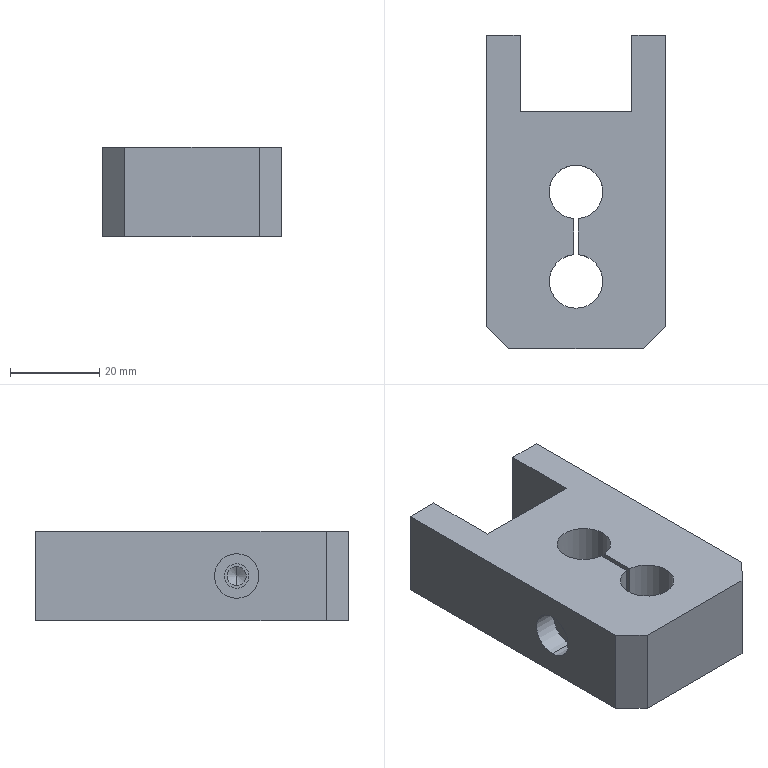Component | SolidWorks | 55-1 | 1 solid | 28 faces | box 40 x 70 x 20 mm | volume 41189 mm3 | plane 15 | cylinder 11 | cone 2 | commonest cylinder face diameters 4.2 x4 12 x3 10 x2 5.5 x2
build123d program:
from build123d import *

# Parameters (mm, degrees)
SKETCH1_W                                            = 20
SKETCH1_H                                            = 80
BOSS_EXTRUDE1_DEPTH                                  = 40
SKETCH2_R                                            = 6
CUT_EXTRUDE1_DEPTH                                   = 40
SKETCH3_W                                            = 1
SKETCH3_H                                            = 21.122
CUT_EXTRUDE2_DEPTH                                   = 40
M5_HEX_SOCKET_HEAD_CAP_SCREW_COUNTERBORE_D           = 5.5
M5_HEX_SOCKET_HEAD_CAP_SCREW_COUNTERBORE_DEPTH       = 19.5
M5_HEX_SOCKET_HEAD_CAP_SCREW_COUNTERBORE_CBORE_D     = 10
M5_HEX_SOCKET_HEAD_CAP_SCREW_COUNTERBORE_CBORE_DEPTH = 5.4
M5_TAPPED_HOLE1_D                                    = 4.2
M5_TAPPED_HOLE1_DEPTH                                = 14
M5_TAPPED_HOLE1_TIP                                  = 1.262
CHAMFER1_SIZE                                        = 5
SKETCH8_W                                            = 25
SKETCH8_H                                            = 27
CUT_EXTRUDE3_DEPTH                                   = 40
M5_TAPPED_HOLE2_D                                    = 4.2
M5_TAPPED_HOLE2_DEPTH                                = 14
M5_TAPPED_HOLE2_TIP                                  = 1.262
SKETCH11_W                                           = 40
SKETCH11_H                                           = 10
CUT_EXTRUDE4_DEPTH                                   = 61


with BuildPart() as part:
    # Sketch1 → Boss-Extrude1 (new body)
    with BuildSketch(Plane.XY):
        Rectangle(SKETCH1_W, SKETCH1_H)
    extrude(amount=BOSS_EXTRUDE1_DEPTH)

    # Sketch2 → Cut-Extrude1 (cut)
    with BuildSketch(Plane.ZY.offset(10)):
        with Locations(Location((20, -5, 0), (0, 0, 270))):
            Circle(SKETCH2_R)
        with Locations(Location((20, -25, 0), (0, 0, 270))):
            Circle(SKETCH2_R)
    extrude(amount=-CUT_EXTRUDE1_DEPTH, mode=Mode.SUBTRACT)

    # Sketch3 → Cut-Extrude2 (cut)
    with BuildSketch(Plane.ZY.offset(10)):
        with Locations((20, -14.461)):
            Rectangle(SKETCH3_W, SKETCH3_H)
    extrude(amount=-CUT_EXTRUDE2_DEPTH, mode=Mode.SUBTRACT)

    # M5 Hex Socket Head Cap Screw Counterbore
    with Locations(Plane.XY.offset(40)):
        with Locations((0, -15)):
            CounterBoreHole(M5_HEX_SOCKET_HEAD_CAP_SCREW_COUNTERBORE_D / 2, M5_HEX_SOCKET_HEAD_CAP_SCREW_COUNTERBORE_CBORE_D / 2, M5_HEX_SOCKET_HEAD_CAP_SCREW_COUNTERBORE_CBORE_DEPTH, depth=M5_HEX_SOCKET_HEAD_CAP_SCREW_COUNTERBORE_DEPTH)

    # M5 Tapped Hole1
    with Locations(Plane.XY.offset(19.5)):
        with Locations((0, -15)):
            Hole(M5_TAPPED_HOLE1_D / 2, depth=M5_TAPPED_HOLE1_DEPTH)
            with Locations((0, 0, -(M5_TAPPED_HOLE1_DEPTH + M5_TAPPED_HOLE1_TIP / 2))):  # 118° drill point
                Cone(0, M5_TAPPED_HOLE1_D / 2, M5_TAPPED_HOLE1_TIP, mode=Mode.SUBTRACT)

    # Chamfer1
    chamfer1_edges = [part.edges().sort_by_distance(p)[0] for p in [
        (0, -40, 0),
        (0, -40, 40),
    ]]
    chamfer(chamfer1_edges, length=CHAMFER1_SIZE)

    # Sketch8 → Cut-Extrude3 (cut)
    with BuildSketch(Plane.ZY.offset(10)):
        with Locations((20, 26.5)):
            Rectangle(SKETCH8_W, SKETCH8_H)
    extrude(amount=-CUT_EXTRUDE3_DEPTH, mode=Mode.SUBTRACT)

    # M5 Tapped Hole2
    with Locations(Plane(origin=(0, 13, 0), x_dir=(1, 0, 0), z_dir=(0, 1, 0))):
        with Locations((0, -20)):
            Hole(M5_TAPPED_HOLE2_D / 2, depth=M5_TAPPED_HOLE2_DEPTH)
            with Locations((0, 0, -(M5_TAPPED_HOLE2_DEPTH + M5_TAPPED_HOLE2_TIP / 2))):  # 118° drill point
                Cone(0, M5_TAPPED_HOLE2_D / 2, M5_TAPPED_HOLE2_TIP, mode=Mode.SUBTRACT)

    # Sketch11 → Cut-Extrude4 (cut, through all)
    with BuildSketch(Plane.ZY.offset(10)):
        with Locations((20, 35)):
            Rectangle(SKETCH11_W, SKETCH11_H)
    extrude(amount=-CUT_EXTRUDE4_DEPTH, mode=Mode.SUBTRACT)


solid = part.part

# Placed as in the assembly
solid = solid.moved(Location((20, -13, 100), (0, -90, 0)))
STEP:
#1=COLOUR_RGB('',0.7922,0.8196,0.9333);
#2=FILL_AREA_STYLE_COLOUR('',#1);
#3=FILL_AREA_STYLE('',(#2));
#4=SURFACE_STYLE_FILL_AREA(#3);
#5=SURFACE_SIDE_STYLE('',(#4));
#6=SURFACE_STYLE_USAGE(.BOTH.,#5);
#7=PRESENTATION_STYLE_ASSIGNMENT((#6));
#8=CARTESIAN_POINT('',(0.08268,-0.4874,3.937));
#9=VERTEX_POINT('',#8);
#10=CARTESIAN_POINT('',(-0.08268,-0.4874,3.937));
#11=VERTEX_POINT('',#10);
#12=CARTESIAN_POINT('',(0.08268,-0.4874,3.937));
#13=CARTESIAN_POINT('',(0.08268,-0.4874,3.932));
#14=CARTESIAN_POINT('',(0.08214,-0.4872,3.926));
#15=CARTESIAN_POINT('',(0.07999,-0.4864,3.915));
#16=CARTESIAN_POINT('',(0.0784,-0.4858,3.91));
#17=CARTESIAN_POINT('',(0.07425,-0.4844,3.9));
#18=CARTESIAN_POINT('',(0.07165,-0.4835,3.895));
#19=CARTESIAN_POINT('',(0.06568,-0.4817,3.887));
#20=CARTESIAN_POINT('',(0.06228,-0.4808,3.882));
#21=CARTESIAN_POINT('',(0.05082,-0.4778,3.871));
#22=CARTESIAN_POINT('',(0.0418,-0.4759,3.865));
#23=CARTESIAN_POINT('',(0.02674,-0.4739,3.859));
#24=CARTESIAN_POINT('',(0.02158,-0.4734,3.857));
#25=CARTESIAN_POINT('',(0.01095,-0.4726,3.855));
#26=CARTESIAN_POINT('',(0.005426,-0.4724,3.854));
#27=CARTESIAN_POINT('',(-0.00547,-0.4724,3.854));
#28=CARTESIAN_POINT('',(-0.01087,-0.4726,3.855));
#29=CARTESIAN_POINT('',(-0.02158,-0.4734,3.857));
#30=CARTESIAN_POINT('',(-0.02683,-0.4739,3.859));
#31=CARTESIAN_POINT('',(-0.04177,-0.4759,3.865));
#32=CARTESIAN_POINT('',(-0.0509,-0.4779,3.871));
#33=CARTESIAN_POINT('',(-0.06227,-0.4808,3.882));
#34=CARTESIAN_POINT('',(-0.06573,-0.4817,3.887));
#35=CARTESIAN_POINT('',(-0.0717,-0.4836,3.895));
#36=CARTESIAN_POINT('',(-0.07424,-0.4844,3.9));
#37=CARTESIAN_POINT('',(-0.07841,-0.4858,3.91));
#38=CARTESIAN_POINT('',(-0.08001,-0.4864,3.915));
#39=CARTESIAN_POINT('',(-0.08213,-0.4872,3.926));
#40=CARTESIAN_POINT('',(-0.08268,-0.4874,3.931));
#41=CARTESIAN_POINT('',(-0.08268,-0.4874,3.937));
#42=B_SPLINE_CURVE_WITH_KNOTS('',3,(#12,#13,#14,#15,#16,#17,#18,#19,#20,#21,#22,#23,#24,#25,#26,#27,#28,#29,#30,#31,#32,#33,#34,#35,#36,#37,#38,#39,#40,#41),.UNSPECIFIED.,.F.,.F.,(4,2,2,2,2,2,2,2,2,2,2,2,2,2,4),(0.006618,0.007032,0.007445,0.007859,0.008272,0.009099,0.009513,0.009926,0.01034,0.01075,0.01158,0.01199,0.01241,0.01282,0.01323),.UNSPECIFIED.);
#43=EDGE_CURVE('',#9,#11,#42,.T.);
#44=ORIENTED_EDGE('',*,*,#43,.F.);
#45=CARTESIAN_POINT('',(0.08268,-0.,3.937));
#46=VERTEX_POINT('',#45);
#47=CARTESIAN_POINT('',(0.08268,-0.,3.937));
#48=DIRECTION('',(0.,1.,-0.));
#49=VECTOR('',#48,39.37);
#50=LINE('',#47,#49);
#51=EDGE_CURVE('',#9,#46,#50,.T.);
#52=ORIENTED_EDGE('',*,*,#51,.T.);
#53=CARTESIAN_POINT('',(-0.08268,-0.,3.937));
#54=VERTEX_POINT('',#53);
#55=CARTESIAN_POINT('',(0.,-0.,3.937));
#56=DIRECTION('',(0.,1.,-0.));
#57=DIRECTION('',(-1.,0.,0.));
#58=AXIS2_PLACEMENT_3D('',#55,#56,#57);
#59=CIRCLE('',#58,0.08268);
#60=EDGE_CURVE('',#46,#54,#59,.T.);
#61=ORIENTED_EDGE('',*,*,#60,.T.);
#62=CARTESIAN_POINT('',(-0.08268,-0.,3.937));
#63=DIRECTION('',(0.,1.,-0.));
#64=VECTOR('',#63,39.37);
#65=LINE('',#62,#64);
#66=EDGE_CURVE('',#11,#54,#65,.T.);
#67=ORIENTED_EDGE('',*,*,#66,.F.);
#68=EDGE_LOOP('',(#44,#52,#61,#67));
#69=FACE_OUTER_BOUND('',#68,.T.);
#70=CARTESIAN_POINT('',(0.,-0.,3.937));
#71=DIRECTION('',(0.,1.,-0.));
#72=DIRECTION('',(-1.,0.,0.));
#73=AXIS2_PLACEMENT_3D('',#70,#71,#72);
#74=CYLINDRICAL_SURFACE('',#73,0.08268);
#75=ADVANCED_FACE('',(#69),#74,.F.);
#76=CARTESIAN_POINT('',(0.5709,-1.102,3.854));
#77=VERTEX_POINT('',#76);
#78=CARTESIAN_POINT('',(0.5709,-1.102,4.02));
#79=VERTEX_POINT('',#78);
#80=CARTESIAN_POINT('',(0.5709,-1.102,3.937));
#81=DIRECTION('',(-1.,0.,0.));
#82=DIRECTION('',(0.,0.,1.));
#83=AXIS2_PLACEMENT_3D('',#80,#81,#82);
#84=CIRCLE('',#83,0.08268);
#85=EDGE_CURVE('',#77,#79,#84,.T.);
#86=ORIENTED_EDGE('',*,*,#85,.F.);
#87=CARTESIAN_POINT('',(0.01969,-1.102,3.854));
#88=VERTEX_POINT('',#87);
#89=CARTESIAN_POINT('',(0.01969,-1.102,3.854));
#90=DIRECTION('',(-1.,0.,0.));
#91=VECTOR('',#90,39.37);
#92=LINE('',#89,#91);
#93=EDGE_CURVE('',#77,#88,#92,.T.);
#94=ORIENTED_EDGE('',*,*,#93,.T.);
#95=CARTESIAN_POINT('',(0.01969,-1.102,4.02));
#96=VERTEX_POINT('',#95);
#97=CARTESIAN_POINT('',(0.01969,-1.102,3.937));
#98=DIRECTION('',(-1.,0.,0.));
#99=DIRECTION('',(0.,0.,1.));
#100=AXIS2_PLACEMENT_3D('',#97,#98,#99);
#101=CIRCLE('',#100,0.08268);
#102=EDGE_CURVE('',#88,#96,#101,.T.);
#103=ORIENTED_EDGE('',*,*,#102,.T.);
#104=CARTESIAN_POINT('',(0.01969,-1.102,4.02));
#105=DIRECTION('',(-1.,0.,0.));
#106=VECTOR('',#105,39.37);
#107=LINE('',#104,#106);
#108=EDGE_CURVE('',#79,#96,#107,.T.);
#109=ORIENTED_EDGE('',*,*,#108,.F.);
#110=EDGE_LOOP('',(#86,#94,#103,#109));
#111=FACE_OUTER_BOUND('',#110,.T.);
#112=CARTESIAN_POINT('',(0.01969,-1.102,3.937));
#113=DIRECTION('',(-1.,0.,0.));
#114=DIRECTION('',(0.,0.,1.));
#115=AXIS2_PLACEMENT_3D('',#112,#113,#114);
#116=CYLINDRICAL_SURFACE('',#115,0.08268);
#117=ADVANCED_FACE('',(#111),#116,.F.);
#118=CARTESIAN_POINT('',(0.6205,-1.102,3.937));
#119=VERTEX_POINT('',#118);
#120=CARTESIAN_POINT('',(0.5709,-1.102,4.02));
#121=DIRECTION('',(-0.515,0.,0.8572));
#122=VECTOR('',#121,39.37);
#123=LINE('',#120,#122);
#124=EDGE_CURVE('',#119,#79,#123,.T.);
#125=ORIENTED_EDGE('',*,*,#124,.F.);
#126=CARTESIAN_POINT('',(0.5709,-1.102,3.854));
#127=DIRECTION('',(-0.515,0.,-0.8572));
#128=VECTOR('',#127,39.37);
#129=LINE('',#126,#128);
#130=EDGE_CURVE('',#119,#77,#129,.T.);
#131=ORIENTED_EDGE('',*,*,#130,.T.);
#132=ORIENTED_EDGE('',*,*,#85,.T.);
#133=EDGE_LOOP('',(#125,#131,#132));
#134=FACE_OUTER_BOUND('',#133,.T.);
#135=CARTESIAN_POINT('',(0.5709,-1.102,3.937));
#136=DIRECTION('',(-1.,0.,0.));
#137=DIRECTION('',(0.,0.,1.));
#138=AXIS2_PLACEMENT_3D('',#135,#136,#137);
#139=CONICAL_SURFACE('',#138,0.08268,1.03);
#140=ADVANCED_FACE('',(#134),#139,.F.);
#141=CARTESIAN_POINT('',(-0.5748,-1.102,3.74));
#142=VERTEX_POINT('',#141);
#143=CARTESIAN_POINT('',(-0.5748,-1.102,4.134));
#144=VERTEX_POINT('',#143);
#145=CARTESIAN_POINT('',(-0.5748,-1.102,3.937));
#146=DIRECTION('',(-1.,0.,0.));
#147=DIRECTION('',(0.,0.,1.));
#148=AXIS2_PLACEMENT_3D('',#145,#146,#147);
#149=CIRCLE('',#148,0.1969);
#150=EDGE_CURVE('',#142,#144,#149,.T.);
#151=ORIENTED_EDGE('',*,*,#150,.F.);
#152=CARTESIAN_POINT('',(-0.7874,-1.102,3.74));
#153=VERTEX_POINT('',#152);
#154=CARTESIAN_POINT('',(-0.7874,-1.102,3.74));
#155=DIRECTION('',(-1.,0.,0.));
#156=VECTOR('',#155,39.37);
#157=LINE('',#154,#156);
#158=EDGE_CURVE('',#142,#153,#157,.T.);
#159=ORIENTED_EDGE('',*,*,#158,.T.);
#160=CARTESIAN_POINT('',(-0.7874,-1.102,4.134));
#161=VERTEX_POINT('',#160);
#162=CARTESIAN_POINT('',(-0.7874,-1.102,3.937));
#163=DIRECTION('',(-1.,0.,0.));
#164=DIRECTION('',(0.,0.,1.));
#165=AXIS2_PLACEMENT_3D('',#162,#163,#164);
#166=CIRCLE('',#165,0.1969);
#167=EDGE_CURVE('',#153,#161,#166,.T.);
#168=ORIENTED_EDGE('',*,*,#167,.T.);
#169=CARTESIAN_POINT('',(-0.7874,-1.102,4.134));
#170=DIRECTION('',(-1.,0.,0.));
#171=VECTOR('',#170,39.37);
#172=LINE('',#169,#171);
#173=EDGE_CURVE('',#144,#161,#172,.T.);
#174=ORIENTED_EDGE('',*,*,#173,.F.);
#175=EDGE_LOOP('',(#151,#159,#168,#174));
#176=FACE_OUTER_BOUND('',#175,.T.);
#177=CARTESIAN_POINT('',(-0.7874,-1.102,3.937));
#178=DIRECTION('',(-1.,0.,0.));
#179=DIRECTION('',(0.,0.,1.));
#180=AXIS2_PLACEMENT_3D('',#177,#178,#179);
#181=CYLINDRICAL_SURFACE('',#180,0.1969);
#182=ADVANCED_FACE('',(#176),#181,.F.);
#183=CARTESIAN_POINT('',(-0.01969,-1.102,3.829));
#184=VERTEX_POINT('',#183);
#185=CARTESIAN_POINT('',(-0.01969,-1.102,4.045));
#186=VERTEX_POINT('',#185);
#187=CARTESIAN_POINT('',(-0.01969,-1.102,3.937));
#188=DIRECTION('',(-1.,0.,-0.));
#189=DIRECTION('',(-0.,-1.,0.));
#190=AXIS2_PLACEMENT_3D('',#187,#188,#189);
#191=CIRCLE('',#190,0.1083);
#192=EDGE_CURVE('',#184,#186,#191,.T.);
#193=ORIENTED_EDGE('',*,*,#192,.F.);
#194=CARTESIAN_POINT('',(-0.5748,-1.102,3.829));
#195=VERTEX_POINT('',#194);
#196=CARTESIAN_POINT('',(-0.7874,-1.102,3.829));
#197=DIRECTION('',(-1.,0.,0.));
#198=VECTOR('',#197,39.37);
#199=LINE('',#196,#198);
#200=EDGE_CURVE('',#184,#195,#199,.T.);
#201=ORIENTED_EDGE('',*,*,#200,.T.);
#202=CARTESIAN_POINT('',(-0.5748,-1.102,4.045));
#203=VERTEX_POINT('',#202);
#204=CARTESIAN_POINT('',(-0.5748,-1.102,3.937));
#205=DIRECTION('',(-1.,0.,0.));
#206=DIRECTION('',(0.,0.,1.));
#207=AXIS2_PLACEMENT_3D('',#204,#205,#206);
#208=CIRCLE('',#207,0.1083);
#209=EDGE_CURVE('',#195,#203,#208,.T.);
#210=ORIENTED_EDGE('',*,*,#209,.T.);
#211=CARTESIAN_POINT('',(-0.7874,-1.102,4.045));
#212=DIRECTION('',(-1.,0.,0.));
#213=VECTOR('',#212,39.37);
#214=LINE('',#211,#213);
#215=EDGE_CURVE('',#186,#203,#214,.T.);
#216=ORIENTED_EDGE('',*,*,#215,.F.);
#217=EDGE_LOOP('',(#193,#201,#210,#216));
#218=FACE_OUTER_BOUND('',#217,.T.);
#219=CARTESIAN_POINT('',(-0.7874,-1.102,3.937));
#220=DIRECTION('',(-1.,0.,0.));
#221=DIRECTION('',(0.,0.,1.));
#222=AXIS2_PLACEMENT_3D('',#219,#220,#221);
#223=CYLINDRICAL_SURFACE('',#222,0.1083);
#224=ADVANCED_FACE('',(#218),#223,.F.);
#225=CARTESIAN_POINT('',(-0.,-1.732,4.331));
#226=VERTEX_POINT('',#225);
#227=CARTESIAN_POINT('',(-0.01969,-1.261,4.331));
#228=VERTEX_POINT('',#227);
#229=CARTESIAN_POINT('',(-0.,-1.496,4.331));
#230=DIRECTION('',(-0.,-0.,-1.));
#231=DIRECTION('',(-0.,-1.,0.));
#232=AXIS2_PLACEMENT_3D('',#229,#230,#231);
#233=CIRCLE('',#232,0.2362);
#234=EDGE_CURVE('',#226,#228,#233,.T.);
#235=ORIENTED_EDGE('',*,*,#234,.F.);
#236=CARTESIAN_POINT('',(-0.,-1.732,3.543));
#237=VERTEX_POINT('',#236);
#238=CARTESIAN_POINT('',(-0.,-1.732,5.118));
#239=DIRECTION('',(-0.,-0.,-1.));
#240=VECTOR('',#239,39.37);
#241=LINE('',#238,#240);
#242=EDGE_CURVE('',#226,#237,#241,.T.);
#243=ORIENTED_EDGE('',*,*,#242,.T.);
#244=CARTESIAN_POINT('',(-0.01969,-1.261,3.543));
#245=VERTEX_POINT('',#244);
#246=CARTESIAN_POINT('',(-0.,-1.496,3.543));
#247=DIRECTION('',(-0.,-0.,-1.));
#248=DIRECTION('',(-0.,-1.,0.));
#249=AXIS2_PLACEMENT_3D('',#246,#247,#248);
#250=CIRCLE('',#249,0.2362);
#251=EDGE_CURVE('',#237,#245,#250,.T.);
#252=ORIENTED_EDGE('',*,*,#251,.T.);
#253=CARTESIAN_POINT('',(-0.01969,-1.261,5.118));
#254=DIRECTION('',(0.,0.,1.));
#255=VECTOR('',#254,39.37);
#256=LINE('',#253,#255);
#257=EDGE_CURVE('',#245,#228,#256,.T.);
#258=ORIENTED_EDGE('',*,*,#257,.T.);
#259=EDGE_LOOP('',(#235,#243,#252,#258));
#260=FACE_OUTER_BOUND('',#259,.T.);
#261=CARTESIAN_POINT('',(-0.,-1.496,5.118));
#262=DIRECTION('',(-0.,-0.,-1.));
#263=DIRECTION('',(-0.,-1.,0.));
#264=AXIS2_PLACEMENT_3D('',#261,#262,#263);
#265=CYLINDRICAL_SURFACE('',#264,0.2362);
#266=ADVANCED_FACE('',(#260),#265,.F.);
#267=CARTESIAN_POINT('',(0.01969,-1.261,3.543));
#268=VERTEX_POINT('',#267);
#269=CARTESIAN_POINT('',(-0.,-1.496,3.543));
#270=DIRECTION('',(-0.,-0.,-1.));
#271=DIRECTION('',(-0.,-1.,0.));
#272=AXIS2_PLACEMENT_3D('',#269,#270,#271);
#273=CIRCLE('',#272,0.2362);
#274=EDGE_CURVE('',#268,#237,#273,.T.);
#275=ORIENTED_EDGE('',*,*,#274,.F.);
#276=CARTESIAN_POINT('',(0.01969,-0.9441,3.543));
#277=VERTEX_POINT('',#276);
#278=CARTESIAN_POINT('',(0.01969,-0.6653,3.543));
#279=DIRECTION('',(-0.,-1.,0.));
#280=VECTOR('',#279,39.37);
#281=LINE('',#278,#280);
#282=EDGE_CURVE('',#277,#268,#281,.T.);
#283=ORIENTED_EDGE('',*,*,#282,.F.);
#284=CARTESIAN_POINT('',(-0.01969,-0.9441,3.543));
#285=VERTEX_POINT('',#284);
#286=CARTESIAN_POINT('',(-0.,-0.7087,3.543));
#287=DIRECTION('',(-0.,-0.,-1.));
#288=DIRECTION('',(-0.,-1.,0.));
#289=AXIS2_PLACEMENT_3D('',#286,#287,#288);
#290=CIRCLE('',#289,0.2362);
#291=EDGE_CURVE('',#285,#277,#290,.T.);
#292=ORIENTED_EDGE('',*,*,#291,.F.);
#293=CARTESIAN_POINT('',(-0.01969,-0.6653,3.543));
#294=DIRECTION('',(0.,1.,-0.));
#295=VECTOR('',#294,39.37);
#296=LINE('',#293,#295);
#297=EDGE_CURVE('',#245,#285,#296,.T.);
#298=ORIENTED_EDGE('',*,*,#297,.F.);
#299=ORIENTED_EDGE('',*,*,#251,.F.);
#300=EDGE_LOOP('',(#275,#283,#292,#298,#299));
#301=FACE_BOUND('',#300,.T.);
#302=CARTESIAN_POINT('',(-0.7874,0.6693,3.543));
#303=VERTEX_POINT('',#302);
#304=CARTESIAN_POINT('',(-0.7874,-1.89,3.543));
#305=VERTEX_POINT('',#304);
#306=CARTESIAN_POINT('',(-0.7874,1.063,3.543));
#307=DIRECTION('',(-0.,-1.,0.));
#308=VECTOR('',#307,39.37);
#309=LINE('',#306,#308);
#310=EDGE_CURVE('',#303,#305,#309,.T.);
#311=ORIENTED_EDGE('',*,*,#310,.F.);
#312=CARTESIAN_POINT('',(-0.4921,0.6693,3.543));
#313=VERTEX_POINT('',#312);
#314=CARTESIAN_POINT('',(0.7874,0.6693,3.543));
#315=DIRECTION('',(-1.,0.,0.));
#316=VECTOR('',#315,39.37);
#317=LINE('',#314,#316);
#318=EDGE_CURVE('',#313,#303,#317,.T.);
#319=ORIENTED_EDGE('',*,*,#318,.F.);
#320=CARTESIAN_POINT('',(-0.4921,-0.,3.543));
#321=VERTEX_POINT('',#320);
#322=CARTESIAN_POINT('',(-0.4921,1.063,3.543));
#323=DIRECTION('',(0.,1.,-0.));
#324=VECTOR('',#323,39.37);
#325=LINE('',#322,#324);
#326=EDGE_CURVE('',#321,#313,#325,.T.);
#327=ORIENTED_EDGE('',*,*,#326,.F.);
#328=CARTESIAN_POINT('',(0.4921,-0.,3.543));
#329=VERTEX_POINT('',#328);
#330=CARTESIAN_POINT('',(0.4921,-0.,3.543));
#331=DIRECTION('',(-1.,0.,0.));
#332=VECTOR('',#331,39.37);
#333=LINE('',#330,#332);
#334=EDGE_CURVE('',#329,#321,#333,.T.);
#335=ORIENTED_EDGE('',*,*,#334,.F.);
#336=CARTESIAN_POINT('',(0.4921,0.6693,3.543));
#337=VERTEX_POINT('',#336);
#338=CARTESIAN_POINT('',(0.4921,1.063,3.543));
#339=DIRECTION('',(-0.,-1.,0.));
#340=VECTOR('',#339,39.37);
#341=LINE('',#338,#340);
#342=EDGE_CURVE('',#337,#329,#341,.T.);
#343=ORIENTED_EDGE('',*,*,#342,.F.);
#344=CARTESIAN_POINT('',(0.7874,0.6693,3.543));
#345=VERTEX_POINT('',#344);
#346=CARTESIAN_POINT('',(0.7874,0.6693,3.543));
#347=DIRECTION('',(-1.,0.,0.));
#348=VECTOR('',#347,39.37);
#349=LINE('',#346,#348);
#350=EDGE_CURVE('',#345,#337,#349,.T.);
#351=ORIENTED_EDGE('',*,*,#350,.F.);
#352=CARTESIAN_POINT('',(0.7874,-1.89,3.543));
#353=VERTEX_POINT('',#352);
#354=CARTESIAN_POINT('',(0.7874,1.063,3.543));
#355=DIRECTION('',(-0.,-1.,0.));
#356=VECTOR('',#355,39.37);
#357=LINE('',#354,#356);
#358=EDGE_CURVE('',#345,#353,#357,.T.);
#359=ORIENTED_EDGE('',*,*,#358,.T.);
#360=CARTESIAN_POINT('',(0.5906,-2.087,3.543));
#361=VERTEX_POINT('',#360);
#362=CARTESIAN_POINT('',(0.5906,-2.087,3.543));
#363=DIRECTION('',(-0.7071,-0.7071,0.));
#364=VECTOR('',#363,39.37);
#365=LINE('',#362,#364);
#366=EDGE_CURVE('',#353,#361,#365,.T.);
#367=ORIENTED_EDGE('',*,*,#366,.T.);
#368=CARTESIAN_POINT('',(-0.5906,-2.087,3.543));
#369=VERTEX_POINT('',#368);
#370=CARTESIAN_POINT('',(-0.7874,-2.087,3.543));
#371=DIRECTION('',(1.,-0.,0.));
#372=VECTOR('',#371,39.37);
#373=LINE('',#370,#372);
#374=EDGE_CURVE('',#369,#361,#373,.T.);
#375=ORIENTED_EDGE('',*,*,#374,.F.);
#376=CARTESIAN_POINT('',(-0.7874,-1.89,3.543));
#377=DIRECTION('',(-0.7071,0.7071,-0.));
#378=VECTOR('',#377,39.37);
#379=LINE('',#376,#378);
#380=EDGE_CURVE('',#369,#305,#379,.T.);
#381=ORIENTED_EDGE('',*,*,#380,.T.);
#382=EDGE_LOOP('',(#311,#319,#327,#335,#343,#351,#359,#367,#375,#381));
#383=FACE_OUTER_BOUND('',#382,.T.);
#384=CARTESIAN_POINT('',(-0.7874,1.063,3.543));
#385=DIRECTION('',(0.,0.,1.));
#386=DIRECTION('',(0.,1.,-0.));
#387=AXIS2_PLACEMENT_3D('',#384,#385,#386);
#388=PLANE('',#387);
#389=ADVANCED_FACE('',(#301,#383),#388,.F.);
#390=ORIENTED_EDGE('',*,*,#374,.T.);
#391=CARTESIAN_POINT('',(0.5906,-2.087,4.331));
#392=VERTEX_POINT('',#391);
#393=CARTESIAN_POINT('',(0.5906,-2.087,3.543));
#394=DIRECTION('',(0.,0.,1.));
#395=VECTOR('',#394,39.37);
#396=LINE('',#393,#395);
#397=EDGE_CURVE('',#361,#392,#396,.T.);
#398=ORIENTED_EDGE('',*,*,#397,.T.);
#399=CARTESIAN_POINT('',(-0.5906,-2.087,4.331));
#400=VERTEX_POINT('',#399);
#401=CARTESIAN_POINT('',(-0.7874,-2.087,4.331));
#402=DIRECTION('',(1.,-0.,0.));
#403=VECTOR('',#402,39.37);
#404=LINE('',#401,#403);
#405=EDGE_CURVE('',#400,#392,#404,.T.);
#406=ORIENTED_EDGE('',*,*,#405,.F.);
#407=CARTESIAN_POINT('',(-0.5906,-2.087,3.543));
#408=DIRECTION('',(-0.,-0.,-1.));
#409=VECTOR('',#408,39.37);
#410=LINE('',#407,#409);
#411=EDGE_CURVE('',#400,#369,#410,.T.);
#412=ORIENTED_EDGE('',*,*,#411,.T.);
#413=EDGE_LOOP('',(#390,#398,#406,#412));
#414=FACE_OUTER_BOUND('',#413,.T.);
#415=CARTESIAN_POINT('',(-0.7874,-2.087,3.543));
#416=DIRECTION('',(0.,1.,-0.));
#417=DIRECTION('',(-1.,0.,0.));
#418=AXIS2_PLACEMENT_3D('',#415,#416,#417);
#419=PLANE('',#418);
#420=ADVANCED_FACE('',(#414),#419,.F.);
#421=CARTESIAN_POINT('',(0.7874,-1.89,4.331));
#422=VERTEX_POINT('',#421);
#423=CARTESIAN_POINT('',(0.7874,0.6693,4.331));
#424=VERTEX_POINT('',#423);
#425=CARTESIAN_POINT('',(0.7874,1.063,4.331));
#426=DIRECTION('',(0.,1.,-0.));
#427=VECTOR('',#426,39.37);
#428=LINE('',#425,#427);
#429=EDGE_CURVE('',#422,#424,#428,.T.);
#430=ORIENTED_EDGE('',*,*,#429,.T.);
#431=CARTESIAN_POINT('',(0.4921,0.6693,4.331));
#432=VERTEX_POINT('',#431);
#433=CARTESIAN_POINT('',(0.7874,0.6693,4.331));
#434=DIRECTION('',(-1.,0.,0.));
#435=VECTOR('',#434,39.37);
#436=LINE('',#433,#435);
#437=EDGE_CURVE('',#424,#432,#436,.T.);
#438=ORIENTED_EDGE('',*,*,#437,.T.);
#439=CARTESIAN_POINT('',(0.4921,-0.,4.331));
#440=VERTEX_POINT('',#439);
#441=CARTESIAN_POINT('',(0.4921,1.063,4.331));
#442=DIRECTION('',(-0.,-1.,0.));
#443=VECTOR('',#442,39.37);
#444=LINE('',#441,#443);
#445=EDGE_CURVE('',#432,#440,#444,.T.);
#446=ORIENTED_EDGE('',*,*,#445,.T.);
#447=CARTESIAN_POINT('',(-0.4921,-0.,4.331));
#448=VERTEX_POINT('',#447);
#449=CARTESIAN_POINT('',(-0.7874,-0.,4.331));
#450=DIRECTION('',(-1.,0.,0.));
#451=VECTOR('',#450,39.37);
#452=LINE('',#449,#451);
#453=EDGE_CURVE('',#440,#448,#452,.T.);
#454=ORIENTED_EDGE('',*,*,#453,.T.);
#455=CARTESIAN_POINT('',(-0.4921,0.6693,4.331));
#456=VERTEX_POINT('',#455);
#457=CARTESIAN_POINT('',(-0.4921,1.063,4.331));
#458=DIRECTION('',(0.,1.,-0.));
#459=VECTOR('',#458,39.37);
#460=LINE('',#457,#459);
#461=EDGE_CURVE('',#448,#456,#460,.T.);
#462=ORIENTED_EDGE('',*,*,#461,.T.);
#463=CARTESIAN_POINT('',(-0.7874,0.6693,4.331));
#464=VERTEX_POINT('',#463);
#465=CARTESIAN_POINT('',(0.7874,0.6693,4.331));
#466=DIRECTION('',(-1.,0.,0.));
#467=VECTOR('',#466,39.37);
#468=LINE('',#465,#467);
#469=EDGE_CURVE('',#456,#464,#468,.T.);
#470=ORIENTED_EDGE('',*,*,#469,.T.);
#471=CARTESIAN_POINT('',(-0.7874,-1.89,4.331));
#472=VERTEX_POINT('',#471);
#473=CARTESIAN_POINT('',(-0.7874,1.063,4.331));
#474=DIRECTION('',(0.,1.,-0.));
#475=VECTOR('',#474,39.37);
#476=LINE('',#473,#475);
#477=EDGE_CURVE('',#472,#464,#476,.T.);
#478=ORIENTED_EDGE('',*,*,#477,.F.);
#479=CARTESIAN_POINT('',(-0.7874,-1.89,4.331));
#480=DIRECTION('',(0.7071,-0.7071,0.));
#481=VECTOR('',#480,39.37);
#482=LINE('',#479,#481);
#483=EDGE_CURVE('',#472,#400,#482,.T.);
#484=ORIENTED_EDGE('',*,*,#483,.T.);
#485=ORIENTED_EDGE('',*,*,#405,.T.);
#486=CARTESIAN_POINT('',(0.5906,-2.087,4.331));
#487=DIRECTION('',(0.7071,0.7071,-0.));
#488=VECTOR('',#487,39.37);
#489=LINE('',#486,#488);
#490=EDGE_CURVE('',#392,#422,#489,.T.);
#491=ORIENTED_EDGE('',*,*,#490,.T.);
#492=EDGE_LOOP('',(#430,#438,#446,#454,#462,#470,#478,#484,#485,#491));
#493=FACE_OUTER_BOUND('',#492,.T.);
#494=CARTESIAN_POINT('',(-0.01969,-0.9441,4.331));
#495=VERTEX_POINT('',#494);
#496=CARTESIAN_POINT('',(0.01969,-0.9441,4.331));
#497=VERTEX_POINT('',#496);
#498=CARTESIAN_POINT('',(-0.,-0.7087,4.331));
#499=DIRECTION('',(-0.,-0.,-1.));
#500=DIRECTION('',(-0.,-1.,0.));
#501=AXIS2_PLACEMENT_3D('',#498,#499,#500);
#502=CIRCLE('',#501,0.2362);
#503=EDGE_CURVE('',#495,#497,#502,.T.);
#504=ORIENTED_EDGE('',*,*,#503,.T.);
#505=CARTESIAN_POINT('',(0.01969,-1.261,4.331));
#506=VERTEX_POINT('',#505);
#507=CARTESIAN_POINT('',(0.01969,1.063,4.331));
#508=DIRECTION('',(-0.,-1.,0.));
#509=VECTOR('',#508,39.37);
#510=LINE('',#507,#509);
#511=EDGE_CURVE('',#497,#506,#510,.T.);
#512=ORIENTED_EDGE('',*,*,#511,.T.);
#513=CARTESIAN_POINT('',(-0.,-1.496,4.331));
#514=DIRECTION('',(-0.,-0.,-1.));
#515=DIRECTION('',(-0.,-1.,0.));
#516=AXIS2_PLACEMENT_3D('',#513,#514,#515);
#517=CIRCLE('',#516,0.2362);
#518=EDGE_CURVE('',#506,#226,#517,.T.);
#519=ORIENTED_EDGE('',*,*,#518,.T.);
#520=ORIENTED_EDGE('',*,*,#234,.T.);
#521=CARTESIAN_POINT('',(-0.01969,1.063,4.331));
#522=DIRECTION('',(0.,1.,-0.));
#523=VECTOR('',#522,39.37);
#524=LINE('',#521,#523);
#525=EDGE_CURVE('',#228,#495,#524,.T.);
#526=ORIENTED_EDGE('',*,*,#525,.T.);
#527=EDGE_LOOP('',(#504,#512,#519,#520,#526));
#528=FACE_BOUND('',#527,.T.);
#529=CARTESIAN_POINT('',(-0.7874,1.063,4.331));
#530=DIRECTION('',(-0.,-0.,-1.));
#531=DIRECTION('',(-0.,-1.,0.));
#532=AXIS2_PLACEMENT_3D('',#529,#530,#531);
#533=PLANE('',#532);
#534=ADVANCED_FACE('',(#493,#528),#533,.F.);
#535=CARTESIAN_POINT('',(-0.7874,0.6693,4.331));
#536=DIRECTION('',(-0.,-0.,-1.));
#537=VECTOR('',#536,39.37);
#538=LINE('',#535,#537);
#539=EDGE_CURVE('',#464,#303,#538,.T.);
#540=ORIENTED_EDGE('',*,*,#539,.T.);
#541=ORIENTED_EDGE('',*,*,#310,.T.);
#542=CARTESIAN_POINT('',(-0.7874,-1.89,4.331));
#543=DIRECTION('',(0.,0.,1.));
#544=VECTOR('',#543,39.37);
#545=LINE('',#542,#544);
#546=EDGE_CURVE('',#305,#472,#545,.T.);
#547=ORIENTED_EDGE('',*,*,#546,.T.);
#548=ORIENTED_EDGE('',*,*,#477,.T.);
#549=EDGE_LOOP('',(#540,#541,#547,#548));
#550=FACE_OUTER_BOUND('',#549,.T.);
#551=CARTESIAN_POINT('',(-0.7874,-1.102,3.937));
#552=DIRECTION('',(-1.,0.,0.));
#553=DIRECTION('',(0.,0.,1.));
#554=AXIS2_PLACEMENT_3D('',#551,#552,#553);
#555=CIRCLE('',#554,0.1969);
#556=EDGE_CURVE('',#161,#153,#555,.T.);
#557=ORIENTED_EDGE('',*,*,#556,.F.);
#558=ORIENTED_EDGE('',*,*,#167,.F.);
#559=EDGE_LOOP('',(#557,#558));
#560=FACE_BOUND('',#559,.T.);
#561=CARTESIAN_POINT('',(-0.7874,-0.5118,3.937));
#562=DIRECTION('',(-1.,0.,0.));
#563=DIRECTION('',(0.,0.,1.));
#564=AXIS2_PLACEMENT_3D('',#561,#562,#563);
#565=PLANE('',#564);
#566=ADVANCED_FACE('',(#550,#560),#565,.T.);
#567=ORIENTED_EDGE('',*,*,#358,.F.);
#568=CARTESIAN_POINT('',(0.7874,0.6693,4.331));
#569=DIRECTION('',(-0.,-0.,-1.));
#570=VECTOR('',#569,39.37);
#571=LINE('',#568,#570);
#572=EDGE_CURVE('',#424,#345,#571,.T.);
#573=ORIENTED_EDGE('',*,*,#572,.F.);
#574=ORIENTED_EDGE('',*,*,#429,.F.);
#575=CARTESIAN_POINT('',(0.7874,-1.89,3.937));
#576=DIRECTION('',(-0.,-0.,-1.));
#577=VECTOR('',#576,39.37);
#578=LINE('',#575,#577);
#579=EDGE_CURVE('',#422,#353,#578,.T.);
#580=ORIENTED_EDGE('',*,*,#579,.T.);
#581=EDGE_LOOP('',(#567,#573,#574,#580));
#582=FACE_OUTER_BOUND('',#581,.T.);
#583=CARTESIAN_POINT('',(0.7874,-0.5118,3.937));
#584=DIRECTION('',(-1.,0.,0.));
#585=DIRECTION('',(0.,0.,1.));
#586=AXIS2_PLACEMENT_3D('',#583,#584,#585);
#587=PLANE('',#586);
#588=ADVANCED_FACE('',(#582),#587,.F.);
#589=CARTESIAN_POINT('',(-0.08268,-0.4874,3.937));
#590=CARTESIAN_POINT('',(-0.08268,-0.4874,3.943));
#591=CARTESIAN_POINT('',(-0.08213,-0.4872,3.948));
#592=CARTESIAN_POINT('',(-0.08,-0.4864,3.959));
#593=CARTESIAN_POINT('',(-0.07839,-0.4858,3.964));
#594=CARTESIAN_POINT('',(-0.07423,-0.4844,3.974));
#595=CARTESIAN_POINT('',(-0.07169,-0.4836,3.979));
#596=CARTESIAN_POINT('',(-0.06569,-0.4817,3.987));
#597=CARTESIAN_POINT('',(-0.06223,-0.4808,3.992));
#598=CARTESIAN_POINT('',(-0.05089,-0.4779,4.003));
#599=CARTESIAN_POINT('',(-0.04174,-0.4759,4.009));
#600=CARTESIAN_POINT('',(-0.02683,-0.4739,4.015));
#601=CARTESIAN_POINT('',(-0.02157,-0.4734,4.017));
#602=CARTESIAN_POINT('',(-0.01088,-0.4726,4.019));
#603=CARTESIAN_POINT('',(-0.005482,-0.4724,4.02));
#604=CARTESIAN_POINT('',(0.005405,-0.4724,4.02));
#605=CARTESIAN_POINT('',(0.01093,-0.4726,4.019));
#606=CARTESIAN_POINT('',(0.02158,-0.4734,4.017));
#607=CARTESIAN_POINT('',(0.02675,-0.4739,4.015));
#608=CARTESIAN_POINT('',(0.03683,-0.4753,4.011));
#609=CARTESIAN_POINT('',(0.04159,-0.4761,4.009));
#610=CARTESIAN_POINT('',(0.0505,-0.4779,4.003));
#611=CARTESIAN_POINT('',(0.05471,-0.4788,3.999));
#612=CARTESIAN_POINT('',(0.0623,-0.4808,3.992));
#613=CARTESIAN_POINT('',(0.06569,-0.4817,3.987));
#614=CARTESIAN_POINT('',(0.07168,-0.4836,3.979));
#615=CARTESIAN_POINT('',(0.07427,-0.4844,3.974));
#616=CARTESIAN_POINT('',(0.07841,-0.4858,3.964));
#617=CARTESIAN_POINT('',(0.07999,-0.4864,3.959));
#618=CARTESIAN_POINT('',(0.08214,-0.4872,3.948));
#619=CARTESIAN_POINT('',(0.08268,-0.4874,3.942));
#620=CARTESIAN_POINT('',(0.08268,-0.4874,3.937));
#621=B_SPLINE_CURVE_WITH_KNOTS('',3,(#589,#590,#591,#592,#593,#594,#595,#596,#597,#598,#599,#600,#601,#602,#603,#604,#605,#606,#607,#608,#609,#610,#611,#612,#613,#614,#615,#616,#617,#618,#619,#620),.UNSPECIFIED.,.F.,.F.,(4,2,2,2,2,2,2,2,2,2,2,2,2,2,2,4),(0.,0.0004136,0.0008273,0.001241,0.001655,0.002482,0.002895,0.003309,0.003723,0.004136,0.00455,0.004964,0.005377,0.005791,0.006205,0.006618),.UNSPECIFIED.);
#622=EDGE_CURVE('',#11,#9,#621,.T.);
#623=ORIENTED_EDGE('',*,*,#622,.T.);
#624=ORIENTED_EDGE('',*,*,#43,.T.);
#625=EDGE_LOOP('',(#623,#624));
#626=FACE_BOUND('',#625,.T.);
#627=ORIENTED_EDGE('',*,*,#291,.T.);
#628=CARTESIAN_POINT('',(0.01969,-0.9441,5.118));
#629=DIRECTION('',(0.,0.,1.));
#630=VECTOR('',#629,39.37);
#631=LINE('',#628,#630);
#632=EDGE_CURVE('',#277,#497,#631,.T.);
#633=ORIENTED_EDGE('',*,*,#632,.T.);
#634=ORIENTED_EDGE('',*,*,#503,.F.);
#635=CARTESIAN_POINT('',(-0.01969,-0.9441,5.118));
#636=DIRECTION('',(-0.,-0.,-1.));
#637=VECTOR('',#636,39.37);
#638=LINE('',#635,#637);
#639=EDGE_CURVE('',#495,#285,#638,.T.);
#640=ORIENTED_EDGE('',*,*,#639,.T.);
#641=EDGE_LOOP('',(#627,#633,#634,#640));
#642=FACE_OUTER_BOUND('',#641,.T.);
#643=CARTESIAN_POINT('',(-0.,-0.7087,5.118));
#644=DIRECTION('',(-0.,-0.,-1.));
#645=DIRECTION('',(-0.,-1.,0.));
#646=AXIS2_PLACEMENT_3D('',#643,#644,#645);
#647=CYLINDRICAL_SURFACE('',#646,0.2362);
#648=ADVANCED_FACE('',(#626,#642),#647,.F.);
#649=ORIENTED_EDGE('',*,*,#242,.F.);
#650=ORIENTED_EDGE('',*,*,#518,.F.);
#651=CARTESIAN_POINT('',(0.01969,-1.261,5.118));
#652=DIRECTION('',(-0.,-0.,-1.));
#653=VECTOR('',#652,39.37);
#654=LINE('',#651,#653);
#655=EDGE_CURVE('',#506,#268,#654,.T.);
#656=ORIENTED_EDGE('',*,*,#655,.T.);
#657=ORIENTED_EDGE('',*,*,#274,.T.);
#658=EDGE_LOOP('',(#649,#650,#656,#657));
#659=FACE_OUTER_BOUND('',#658,.T.);
#660=CARTESIAN_POINT('',(-0.,-1.496,5.118));
#661=DIRECTION('',(-0.,-0.,-1.));
#662=DIRECTION('',(-0.,-1.,0.));
#663=AXIS2_PLACEMENT_3D('',#660,#661,#662);
#664=CYLINDRICAL_SURFACE('',#663,0.2362);
#665=ADVANCED_FACE('',(#659),#664,.F.);
#666=CARTESIAN_POINT('',(-0.01969,-1.102,3.937));
#667=DIRECTION('',(-1.,0.,-0.));
#668=DIRECTION('',(-0.,-1.,0.));
#669=AXIS2_PLACEMENT_3D('',#666,#667,#668);
#670=CIRCLE('',#669,0.1083);
#671=EDGE_CURVE('',#186,#184,#670,.T.);
#672=ORIENTED_EDGE('',*,*,#671,.T.);
#673=ORIENTED_EDGE('',*,*,#192,.T.);
#674=EDGE_LOOP('',(#672,#673));
#675=FACE_BOUND('',#674,.T.);
#676=ORIENTED_EDGE('',*,*,#525,.F.);
#677=ORIENTED_EDGE('',*,*,#257,.F.);
#678=ORIENTED_EDGE('',*,*,#297,.T.);
#679=ORIENTED_EDGE('',*,*,#639,.F.);
#680=EDGE_LOOP('',(#676,#677,#678,#679));
#681=FACE_OUTER_BOUND('',#680,.T.);
#682=CARTESIAN_POINT('',(-0.01969,-0.6653,5.118));
#683=DIRECTION('',(-1.,0.,-0.));
#684=DIRECTION('',(-0.,-1.,0.));
#685=AXIS2_PLACEMENT_3D('',#682,#683,#684);
#686=PLANE('',#685);
#687=ADVANCED_FACE('',(#675,#681),#686,.F.);
#688=CARTESIAN_POINT('',(0.01969,-1.102,3.937));
#689=DIRECTION('',(-1.,0.,0.));
#690=DIRECTION('',(0.,0.,1.));
#691=AXIS2_PLACEMENT_3D('',#688,#689,#690);
#692=CIRCLE('',#691,0.08268);
#693=EDGE_CURVE('',#96,#88,#692,.T.);
#694=ORIENTED_EDGE('',*,*,#693,.F.);
#695=ORIENTED_EDGE('',*,*,#102,.F.);
#696=EDGE_LOOP('',(#694,#695));
#697=FACE_BOUND('',#696,.T.);
#698=ORIENTED_EDGE('',*,*,#282,.T.);
#699=ORIENTED_EDGE('',*,*,#655,.F.);
#700=ORIENTED_EDGE('',*,*,#511,.F.);
#701=ORIENTED_EDGE('',*,*,#632,.F.);
#702=EDGE_LOOP('',(#698,#699,#700,#701));
#703=FACE_OUTER_BOUND('',#702,.T.);
#704=CARTESIAN_POINT('',(0.01969,-0.6653,5.118));
#705=DIRECTION('',(1.,-0.,0.));
#706=DIRECTION('',(0.,1.,-0.));
#707=AXIS2_PLACEMENT_3D('',#704,#705,#706);
#708=PLANE('',#707);
#709=ADVANCED_FACE('',(#697,#703),#708,.F.);
#710=ORIENTED_EDGE('',*,*,#200,.F.);
#711=ORIENTED_EDGE('',*,*,#671,.F.);
#712=ORIENTED_EDGE('',*,*,#215,.T.);
#713=CARTESIAN_POINT('',(-0.5748,-1.102,3.937));
#714=DIRECTION('',(-1.,0.,0.));
#715=DIRECTION('',(0.,0.,1.));
#716=AXIS2_PLACEMENT_3D('',#713,#714,#715);
#717=CIRCLE('',#716,0.1083);
#718=EDGE_CURVE('',#203,#195,#717,.T.);
#719=ORIENTED_EDGE('',*,*,#718,.T.);
#720=EDGE_LOOP('',(#710,#711,#712,#719));
#721=FACE_OUTER_BOUND('',#720,.T.);
#722=CARTESIAN_POINT('',(-0.7874,-1.102,3.937));
#723=DIRECTION('',(-1.,0.,0.));
#724=DIRECTION('',(0.,0.,1.));
#725=AXIS2_PLACEMENT_3D('',#722,#723,#724);
#726=CYLINDRICAL_SURFACE('',#725,0.1083);
#727=ADVANCED_FACE('',(#721),#726,.F.);
#728=ORIENTED_EDGE('',*,*,#718,.F.);
#729=ORIENTED_EDGE('',*,*,#209,.F.);
#730=EDGE_LOOP('',(#728,#729));
#731=FACE_BOUND('',#730,.T.);
#732=CARTESIAN_POINT('',(-0.5748,-1.102,3.937));
#733=DIRECTION('',(-1.,0.,0.));
#734=DIRECTION('',(0.,0.,1.));
#735=AXIS2_PLACEMENT_3D('',#732,#733,#734);
#736=CIRCLE('',#735,0.1969);
#737=EDGE_CURVE('',#144,#142,#736,.T.);
#738=ORIENTED_EDGE('',*,*,#737,.T.);
#739=ORIENTED_EDGE('',*,*,#150,.T.);
#740=EDGE_LOOP('',(#738,#739));
#741=FACE_OUTER_BOUND('',#740,.T.);
#742=CARTESIAN_POINT('',(-0.5748,-1.102,4.045));
#743=DIRECTION('',(1.,-0.,0.));
#744=DIRECTION('',(-0.,-0.,-1.));
#745=AXIS2_PLACEMENT_3D('',#742,#743,#744);
#746=PLANE('',#745);
#747=ADVANCED_FACE('',(#731,#741),#746,.F.);
#748=ORIENTED_EDGE('',*,*,#158,.F.);
#749=ORIENTED_EDGE('',*,*,#737,.F.);
#750=ORIENTED_EDGE('',*,*,#173,.T.);
#751=ORIENTED_EDGE('',*,*,#556,.T.);
#752=EDGE_LOOP('',(#748,#749,#750,#751));
#753=FACE_OUTER_BOUND('',#752,.T.);
#754=CARTESIAN_POINT('',(-0.7874,-1.102,3.937));
#755=DIRECTION('',(-1.,0.,0.));
#756=DIRECTION('',(0.,0.,1.));
#757=AXIS2_PLACEMENT_3D('',#754,#755,#756);
#758=CYLINDRICAL_SURFACE('',#757,0.1969);
#759=ADVANCED_FACE('',(#753),#758,.F.);
#760=ORIENTED_EDGE('',*,*,#130,.F.);
#761=ORIENTED_EDGE('',*,*,#124,.T.);
#762=CARTESIAN_POINT('',(0.5709,-1.102,3.937));
#763=DIRECTION('',(-1.,0.,0.));
#764=DIRECTION('',(0.,0.,1.));
#765=AXIS2_PLACEMENT_3D('',#762,#763,#764);
#766=CIRCLE('',#765,0.08268);
#767=EDGE_CURVE('',#79,#77,#766,.T.);
#768=ORIENTED_EDGE('',*,*,#767,.T.);
#769=EDGE_LOOP('',(#760,#761,#768));
#770=FACE_OUTER_BOUND('',#769,.T.);
#771=CARTESIAN_POINT('',(0.5709,-1.102,3.937));
#772=DIRECTION('',(-1.,0.,0.));
#773=DIRECTION('',(0.,0.,1.));
#774=AXIS2_PLACEMENT_3D('',#771,#772,#773);
#775=CONICAL_SURFACE('',#774,0.08268,1.03);
#776=ADVANCED_FACE('',(#770),#775,.F.);
#777=ORIENTED_EDGE('',*,*,#93,.F.);
#778=ORIENTED_EDGE('',*,*,#767,.F.);
#779=ORIENTED_EDGE('',*,*,#108,.T.);
#780=ORIENTED_EDGE('',*,*,#693,.T.);
#781=EDGE_LOOP('',(#777,#778,#779,#780));
#782=FACE_OUTER_BOUND('',#781,.T.);
#783=CARTESIAN_POINT('',(0.01969,-1.102,3.937));
#784=DIRECTION('',(-1.,0.,0.));
#785=DIRECTION('',(0.,0.,1.));
#786=AXIS2_PLACEMENT_3D('',#783,#784,#785);
#787=CYLINDRICAL_SURFACE('',#786,0.08268);
#788=ADVANCED_FACE('',(#782),#787,.F.);
#789=ORIENTED_EDGE('',*,*,#366,.F.);
#790=ORIENTED_EDGE('',*,*,#579,.F.);
#791=ORIENTED_EDGE('',*,*,#490,.F.);
#792=ORIENTED_EDGE('',*,*,#397,.F.);
#793=EDGE_LOOP('',(#789,#790,#791,#792));
#794=FACE_OUTER_BOUND('',#793,.T.);
#795=CARTESIAN_POINT('',(0.5906,-2.087,3.543));
#796=DIRECTION('',(-0.7071,0.7071,-0.));
#797=DIRECTION('',(0.,0.,1.));
#798=AXIS2_PLACEMENT_3D('',#795,#796,#797);
#799=PLANE('',#798);
#800=ADVANCED_FACE('',(#794),#799,.F.);
#801=ORIENTED_EDGE('',*,*,#380,.F.);
#802=ORIENTED_EDGE('',*,*,#411,.F.);
#803=ORIENTED_EDGE('',*,*,#483,.F.);
#804=ORIENTED_EDGE('',*,*,#546,.F.);
#805=EDGE_LOOP('',(#801,#802,#803,#804));
#806=FACE_OUTER_BOUND('',#805,.T.);
#807=CARTESIAN_POINT('',(-0.7874,-1.89,3.937));
#808=DIRECTION('',(-0.7071,-0.7071,0.));
#809=DIRECTION('',(-0.,-0.,-1.));
#810=AXIS2_PLACEMENT_3D('',#807,#808,#809);
#811=PLANE('',#810);
#812=ADVANCED_FACE('',(#806),#811,.T.);
#813=CARTESIAN_POINT('',(0.,-0.,3.937));
#814=DIRECTION('',(0.,1.,-0.));
#815=DIRECTION('',(-1.,0.,0.));
#816=AXIS2_PLACEMENT_3D('',#813,#814,#815);
#817=CIRCLE('',#816,0.08268);
#818=EDGE_CURVE('',#54,#46,#817,.T.);
#819=ORIENTED_EDGE('',*,*,#818,.F.);
#820=ORIENTED_EDGE('',*,*,#60,.F.);
#821=EDGE_LOOP('',(#819,#820));
#822=FACE_BOUND('',#821,.T.);
#823=CARTESIAN_POINT('',(0.4921,-0.,5.118));
#824=DIRECTION('',(-0.,-0.,-1.));
#825=VECTOR('',#824,39.37);
#826=LINE('',#823,#825);
#827=EDGE_CURVE('',#440,#329,#826,.T.);
#828=ORIENTED_EDGE('',*,*,#827,.T.);
#829=ORIENTED_EDGE('',*,*,#334,.T.);
#830=CARTESIAN_POINT('',(-0.4921,0.,5.118));
#831=DIRECTION('',(-0.,-0.,-1.));
#832=VECTOR('',#831,39.37);
#833=LINE('',#830,#832);
#834=EDGE_CURVE('',#448,#321,#833,.T.);
#835=ORIENTED_EDGE('',*,*,#834,.F.);
#836=ORIENTED_EDGE('',*,*,#453,.F.);
#837=EDGE_LOOP('',(#828,#829,#835,#836));
#838=FACE_OUTER_BOUND('',#837,.T.);
#839=CARTESIAN_POINT('',(0.4921,-0.,5.118));
#840=DIRECTION('',(-0.,-1.,0.));
#841=DIRECTION('',(0.,0.,1.));
#842=AXIS2_PLACEMENT_3D('',#839,#840,#841);
#843=PLANE('',#842);
#844=ADVANCED_FACE('',(#822,#838),#843,.F.);
#845=ORIENTED_EDGE('',*,*,#445,.F.);
#846=CARTESIAN_POINT('',(0.4921,0.6693,5.118));
#847=DIRECTION('',(-0.,-0.,-1.));
#848=VECTOR('',#847,39.37);
#849=LINE('',#846,#848);
#850=EDGE_CURVE('',#432,#337,#849,.T.);
#851=ORIENTED_EDGE('',*,*,#850,.T.);
#852=ORIENTED_EDGE('',*,*,#342,.T.);
#853=ORIENTED_EDGE('',*,*,#827,.F.);
#854=EDGE_LOOP('',(#845,#851,#852,#853));
#855=FACE_OUTER_BOUND('',#854,.T.);
#856=CARTESIAN_POINT('',(0.4921,1.063,5.118));
#857=DIRECTION('',(1.,-0.,0.));
#858=DIRECTION('',(0.,1.,-0.));
#859=AXIS2_PLACEMENT_3D('',#856,#857,#858);
#860=PLANE('',#859);
#861=ADVANCED_FACE('',(#855),#860,.F.);
#862=ORIENTED_EDGE('',*,*,#326,.T.);
#863=CARTESIAN_POINT('',(-0.4921,0.6693,5.118));
#864=DIRECTION('',(0.,0.,1.));
#865=VECTOR('',#864,39.37);
#866=LINE('',#863,#865);
#867=EDGE_CURVE('',#313,#456,#866,.T.);
#868=ORIENTED_EDGE('',*,*,#867,.T.);
#869=ORIENTED_EDGE('',*,*,#461,.F.);
#870=ORIENTED_EDGE('',*,*,#834,.T.);
#871=EDGE_LOOP('',(#862,#868,#869,#870));
#872=FACE_OUTER_BOUND('',#871,.T.);
#873=CARTESIAN_POINT('',(-0.4921,1.063,5.118));
#874=DIRECTION('',(-1.,0.,0.));
#875=DIRECTION('',(0.,0.,1.));
#876=AXIS2_PLACEMENT_3D('',#873,#874,#875);
#877=PLANE('',#876);
#878=ADVANCED_FACE('',(#872),#877,.F.);
#879=ORIENTED_EDGE('',*,*,#51,.F.);
#880=ORIENTED_EDGE('',*,*,#622,.F.);
#881=ORIENTED_EDGE('',*,*,#66,.T.);
#882=ORIENTED_EDGE('',*,*,#818,.T.);
#883=EDGE_LOOP('',(#879,#880,#881,#882));
#884=FACE_OUTER_BOUND('',#883,.T.);
#885=CARTESIAN_POINT('',(0.,-0.,3.937));
#886=DIRECTION('',(0.,1.,-0.));
#887=DIRECTION('',(-1.,0.,0.));
#888=AXIS2_PLACEMENT_3D('',#885,#886,#887);
#889=CYLINDRICAL_SURFACE('',#888,0.08268);
#890=ADVANCED_FACE('',(#884),#889,.F.);
#891=ORIENTED_EDGE('',*,*,#318,.T.);
#892=ORIENTED_EDGE('',*,*,#539,.F.);
#893=ORIENTED_EDGE('',*,*,#469,.F.);
#894=ORIENTED_EDGE('',*,*,#867,.F.);
#895=EDGE_LOOP('',(#891,#892,#893,#894));
#896=FACE_OUTER_BOUND('',#895,.T.);
#897=CARTESIAN_POINT('',(0.7874,0.6693,4.331));
#898=DIRECTION('',(-0.,-1.,0.));
#899=DIRECTION('',(0.,0.,1.));
#900=AXIS2_PLACEMENT_3D('',#897,#898,#899);
#901=PLANE('',#900);
#902=ADVANCED_FACE('',(#896),#901,.F.);
#903=ORIENTED_EDGE('',*,*,#437,.F.);
#904=ORIENTED_EDGE('',*,*,#572,.T.);
#905=ORIENTED_EDGE('',*,*,#350,.T.);
#906=ORIENTED_EDGE('',*,*,#850,.F.);
#907=EDGE_LOOP('',(#903,#904,#905,#906));
#908=FACE_OUTER_BOUND('',#907,.T.);
#909=CARTESIAN_POINT('',(0.7874,0.6693,4.331));
#910=DIRECTION('',(-0.,-1.,0.));
#911=DIRECTION('',(0.,0.,1.));
#912=AXIS2_PLACEMENT_3D('',#909,#910,#911);
#913=PLANE('',#912);
#914=ADVANCED_FACE('',(#908),#913,.F.);
#915=CLOSED_SHELL('',(#75,#117,#140,#182,#224,#266,#389,#420,#534,#566,#588,#648,#665,#687,#709,#727,#747,#759,#776,#788,#800,#812,#844,#861,#878,#890,#902,#914));
#916=MANIFOLD_SOLID_BREP('',#915);
#917=STYLED_ITEM('',(#7),#916);
#918=(LENGTH_UNIT()NAMED_UNIT(*)SI_UNIT($,.METRE.));
#919=LENGTH_MEASURE_WITH_UNIT(LENGTH_MEASURE(0.0254),#918);
#920=DIMENSIONAL_EXPONENTS(1.,0.,0.,0.,0.,0.,0.);
#921=(CONVERSION_BASED_UNIT('',#919)LENGTH_UNIT()NAMED_UNIT(#920));
#922=UNCERTAINTY_MEASURE_WITH_UNIT(LENGTH_MEASURE(0.00001),#921,'','');
#923=(NAMED_UNIT(*)PLANE_ANGLE_UNIT()SI_UNIT($,.RADIAN.));
#924=(NAMED_UNIT(*)SI_UNIT($,.STERADIAN.)SOLID_ANGLE_UNIT());
#925=(GEOMETRIC_REPRESENTATION_CONTEXT(3)GLOBAL_UNCERTAINTY_ASSIGNED_CONTEXT((#922))GLOBAL_UNIT_ASSIGNED_CONTEXT((#921,#923,#924))REPRESENTATION_CONTEXT('',''));
#926=MECHANICAL_DESIGN_GEOMETRIC_PRESENTATION_REPRESENTATION('',(#917),#925);
#927=CARTESIAN_POINT('',(0.,0.,0.));
#928=DIRECTION('',(0.,0.,1.));
#929=DIRECTION('',(1.,0.,0.));
#930=AXIS2_PLACEMENT_3D('',#927,#928,#929);
#931=(LENGTH_UNIT()NAMED_UNIT(*)SI_UNIT($,.METRE.));
#932=LENGTH_MEASURE_WITH_UNIT(LENGTH_MEASURE(0.0254),#931);
#933=DIMENSIONAL_EXPONENTS(1.,0.,0.,0.,0.,0.,0.);
#934=(CONVERSION_BASED_UNIT('',#932)LENGTH_UNIT()NAMED_UNIT(#933));
#935=UNCERTAINTY_MEASURE_WITH_UNIT(LENGTH_MEASURE(0.00001),#934,'','');
#936=(NAMED_UNIT(*)PLANE_ANGLE_UNIT()SI_UNIT($,.RADIAN.));
#937=(NAMED_UNIT(*)SI_UNIT($,.STERADIAN.)SOLID_ANGLE_UNIT());
#938=(GEOMETRIC_REPRESENTATION_CONTEXT(3)GLOBAL_UNCERTAINTY_ASSIGNED_CONTEXT((#935))GLOBAL_UNIT_ASSIGNED_CONTEXT((#934,#936,#937))REPRESENTATION_CONTEXT('',''));
#939=ADVANCED_BREP_SHAPE_REPRESENTATION('',(#916,#930),#938);
#940=PRESENTATION_LAYER_ASSIGNMENT('','',(#917));